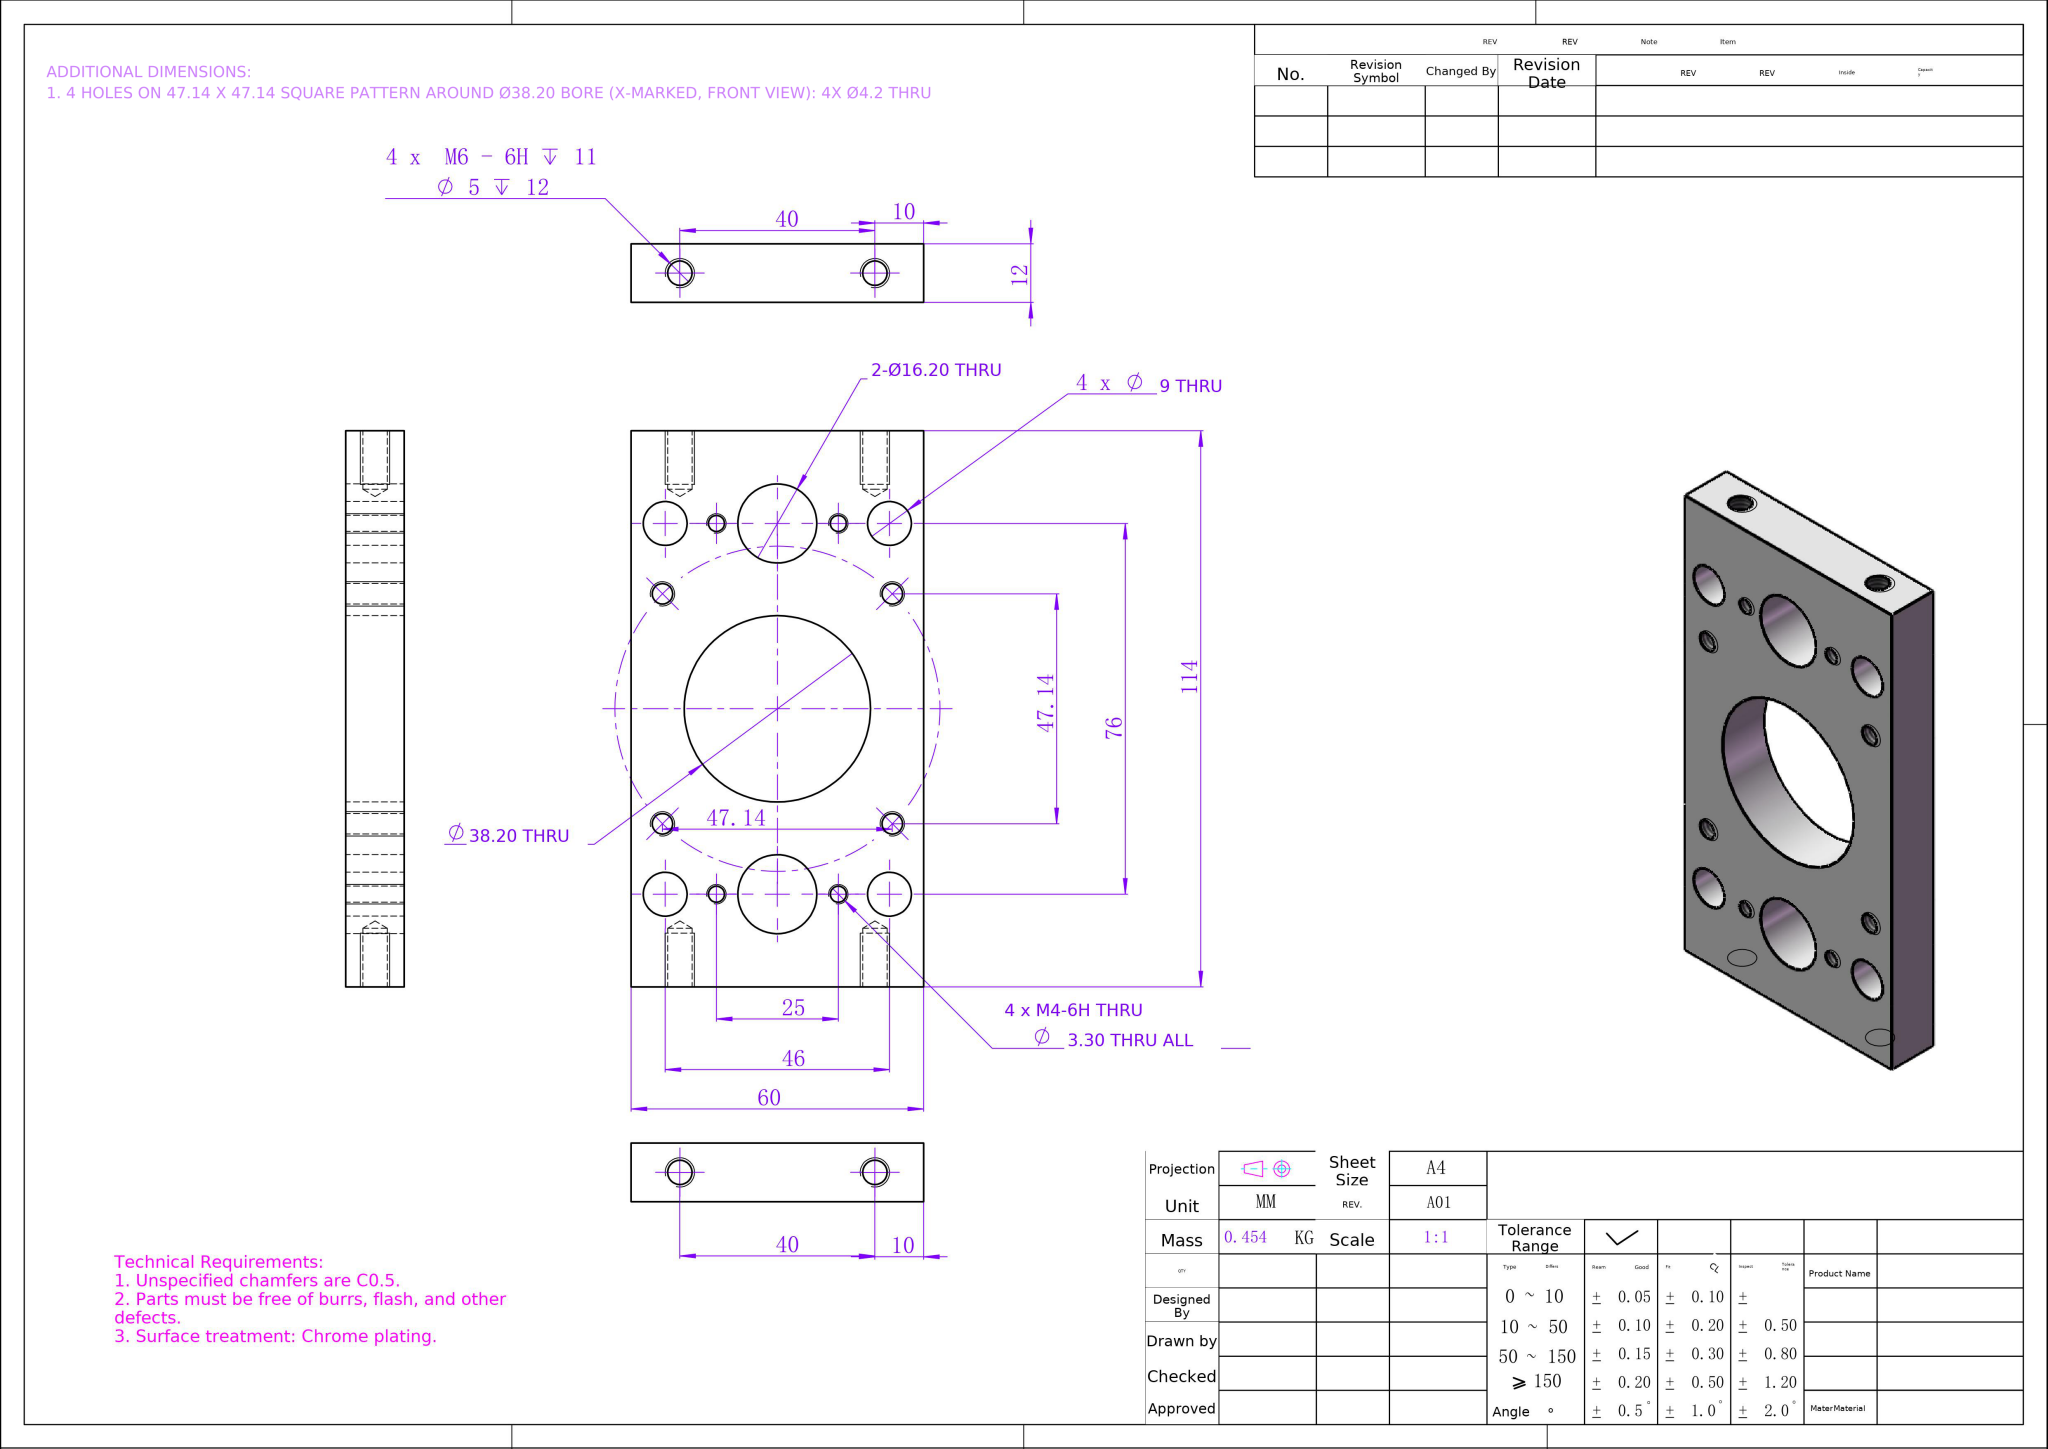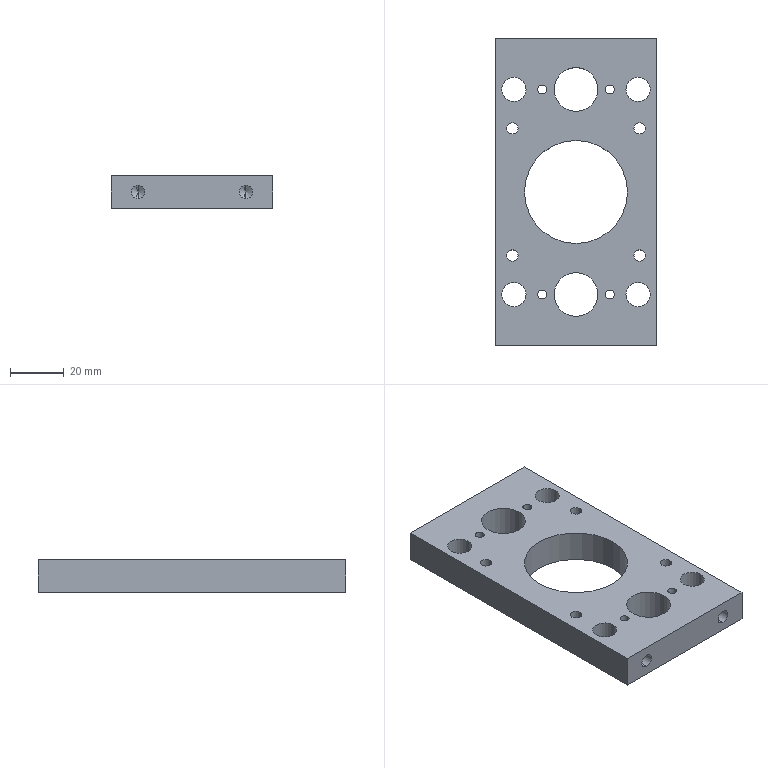Part | NX | mm | 1 solid | 52 faces | box 60 x 114 x 12 mm | volume 58269 mm3 | cylinder 38 | cone 8 | plane 6 | commonest cylinder face diameters 4.2 x8 9 x8 3.3 x8 5 x8 16.2 x4 38.2 x2